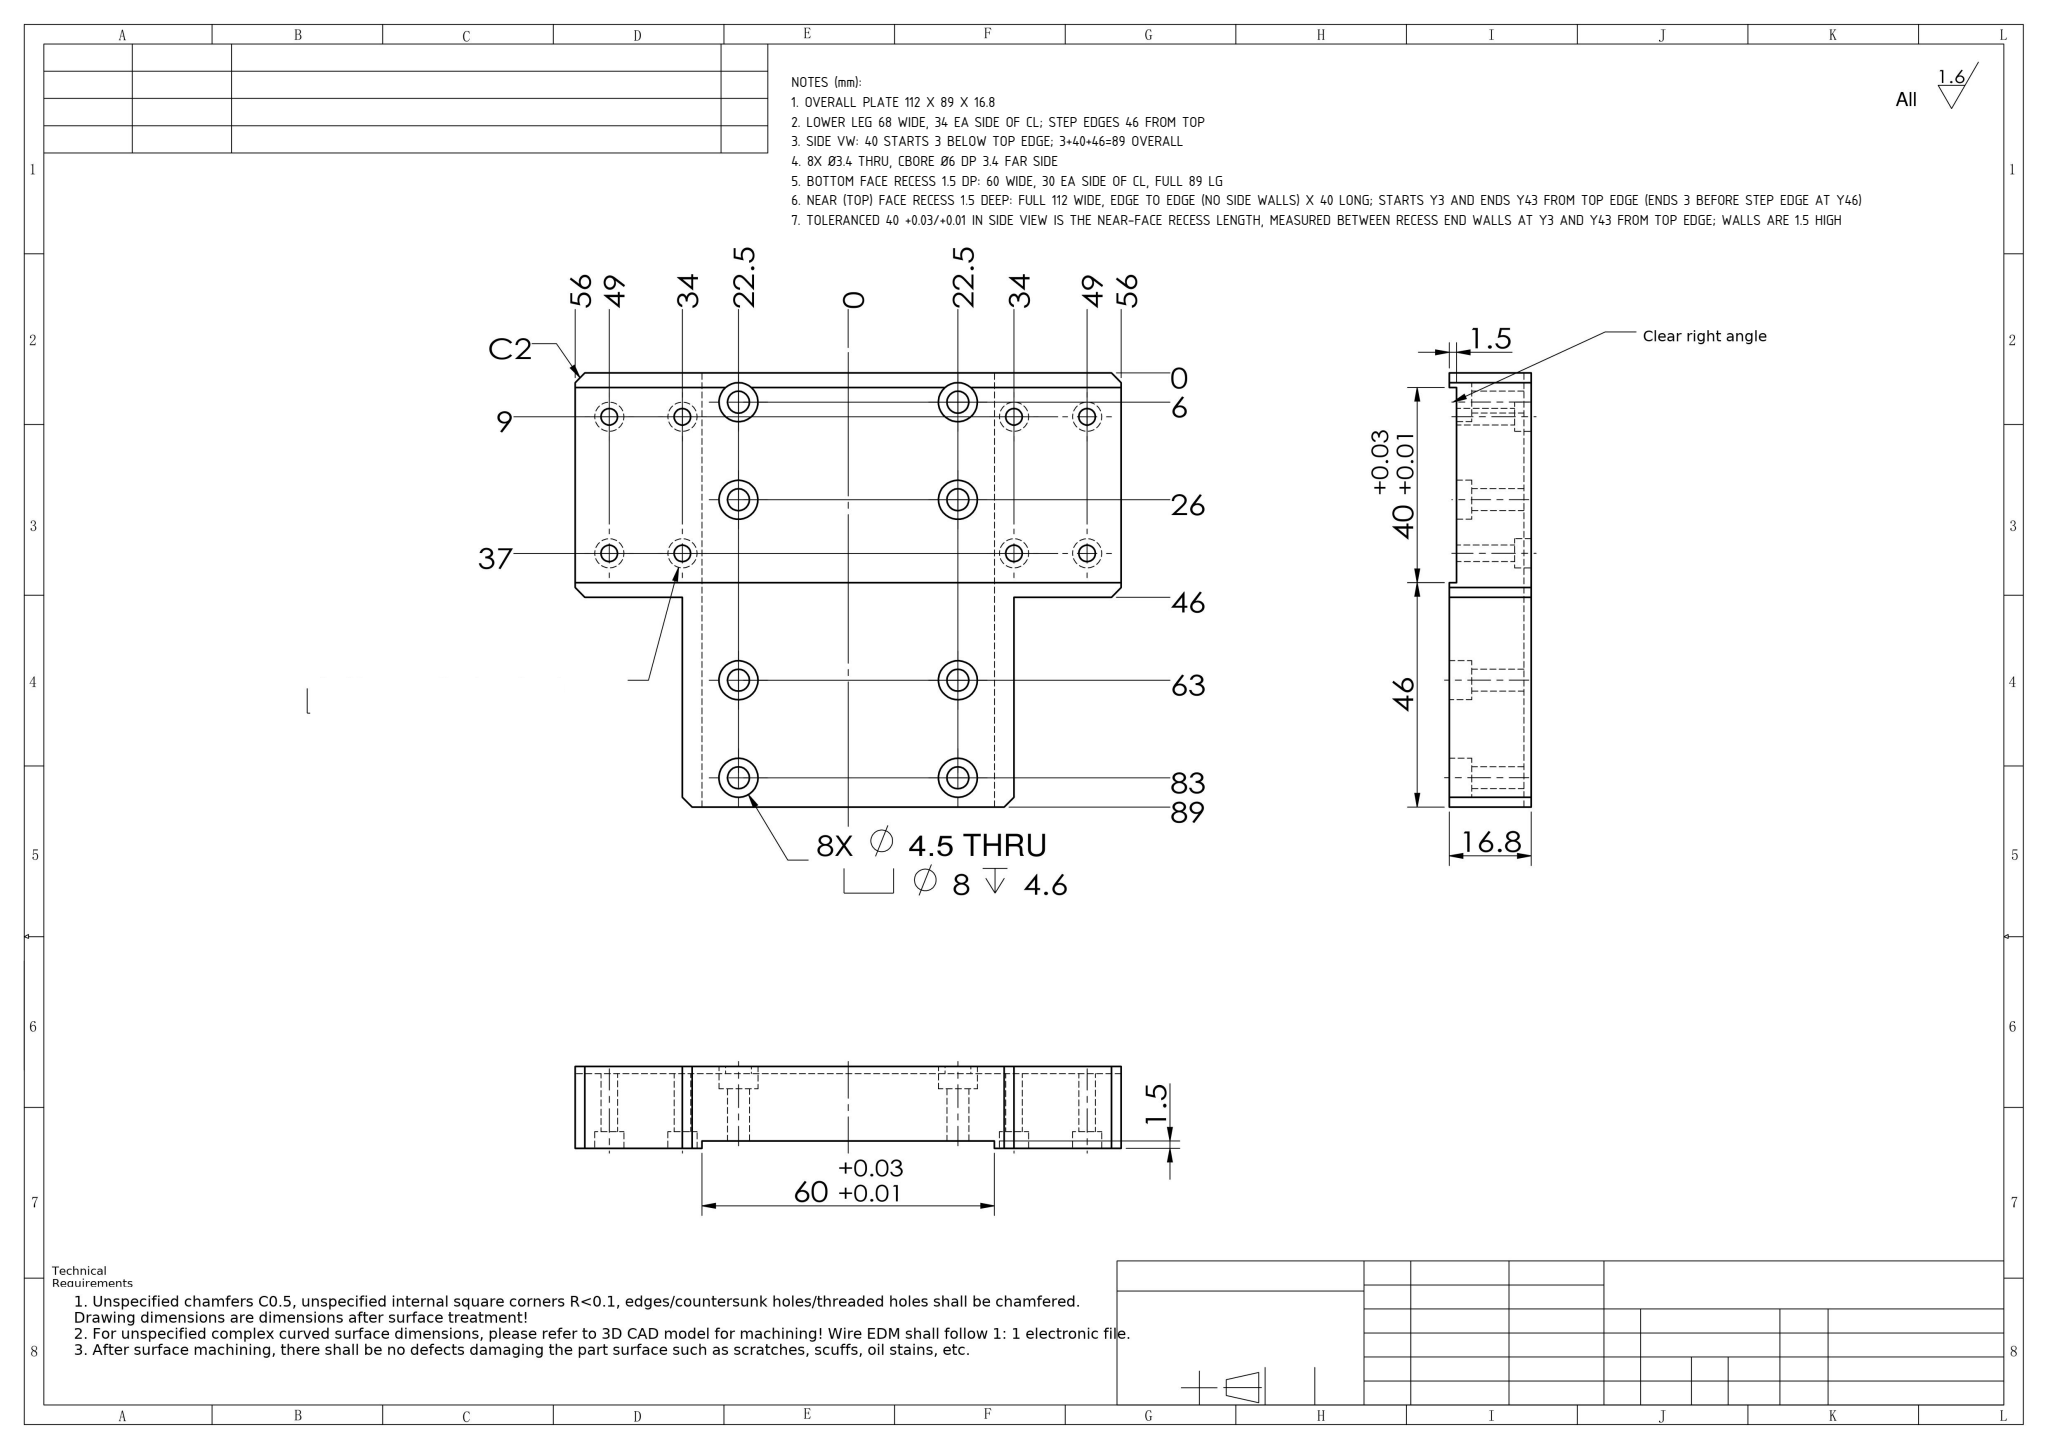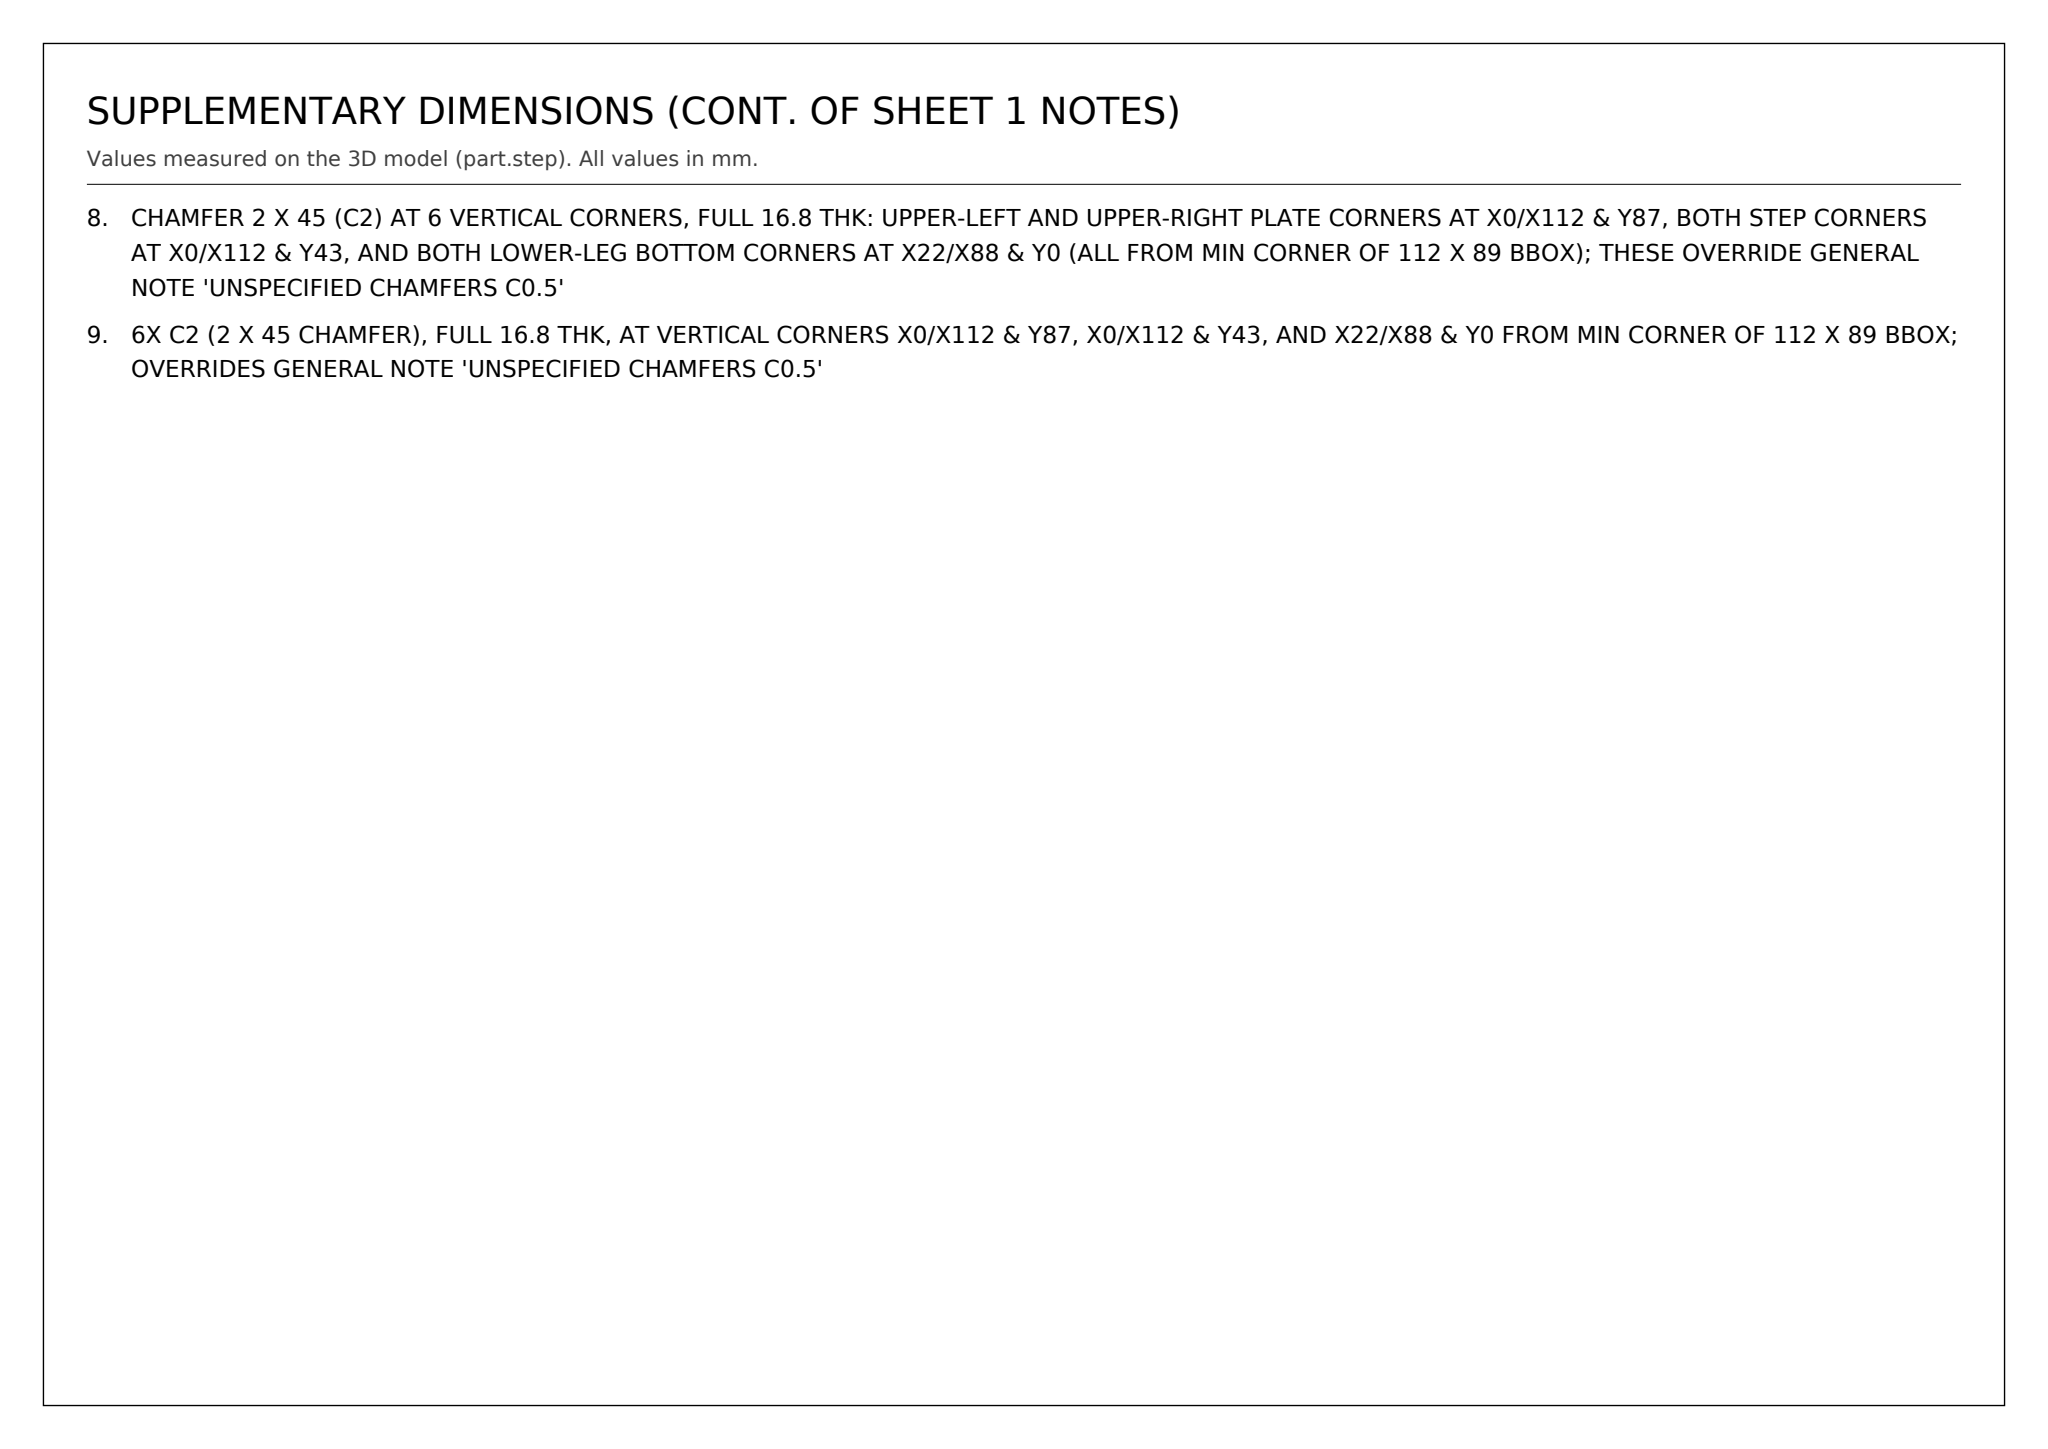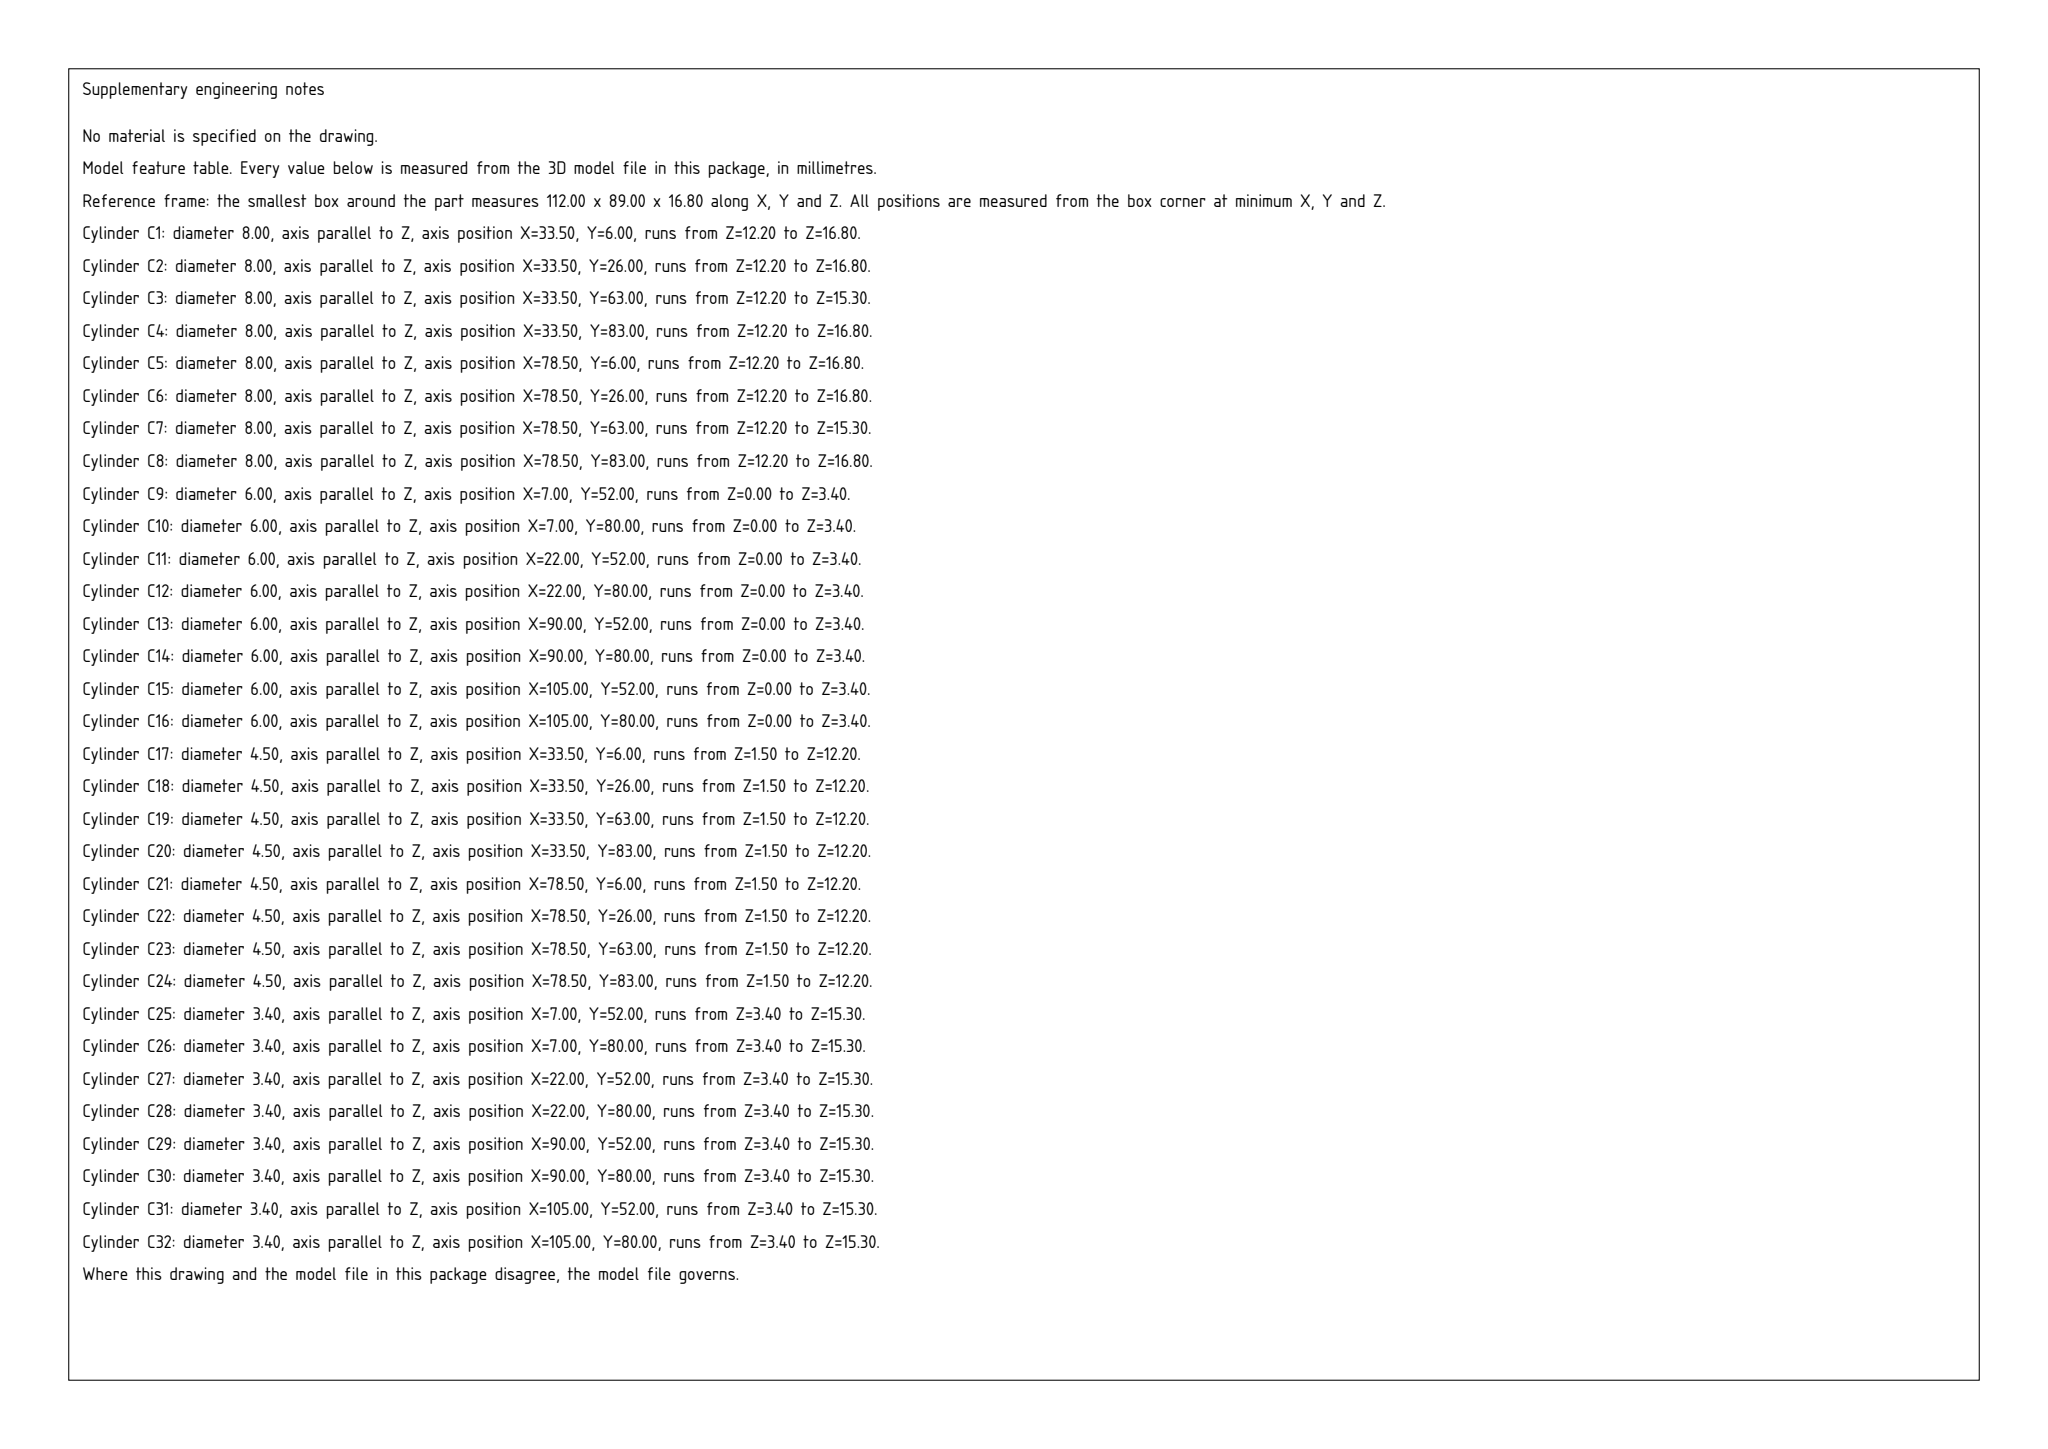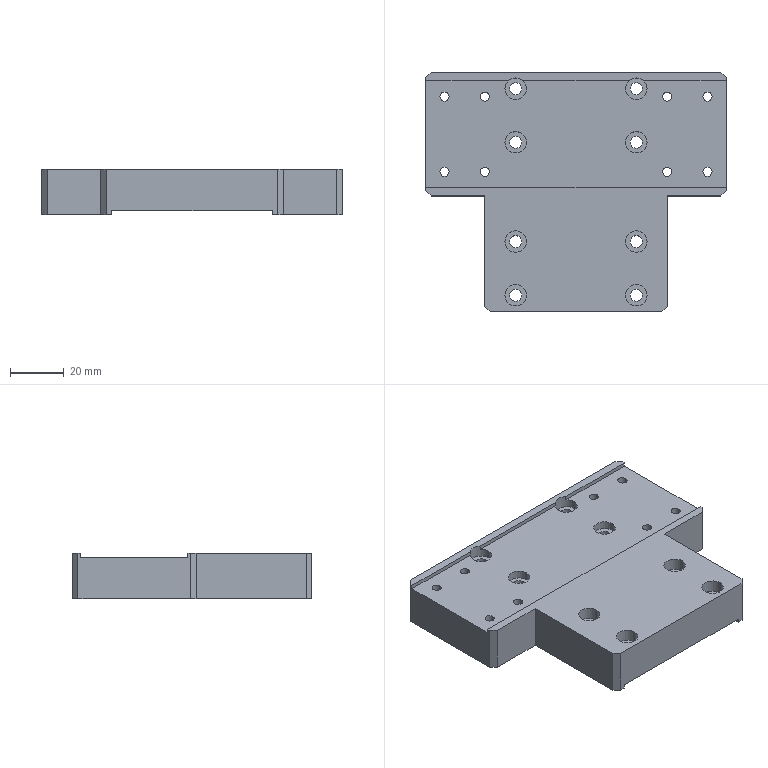Part | SolidWorks | mm | 1 solid | 106 faces | box 112 x 89 x 16.8 mm | volume 116191 mm3 | cylinder 64 | plane 42 | commonest cylinder face diameters 6 x16 3.4 x16 8 x16 4.5 x16
Drawing notes:
OVERALL PLATE 112 X 89 X 16.8 | from the solid: bbox_xyz [112.0, 89.0, 16.8]
LOWER LEG 68 WIDE, 34 EA SIDE OF CL; STEP EDGES 46 FROM TOP | from the solid: Leg side faces are planes x=22.0 and x=90.0, each spanning y[2,43] over full z[0,16.8] -> leg width 90-22 = 68, symmetric about CL at x=56 (34 each side). Step walls are planes y=43 at x[2,22] and x[90,110], i.e. 89-43 = 46 from the top edge.
SIDE VW: 40 STARTS 3 BELOW TOP EDGE; 3+40+46=89 OVERALL | from the solid: y-planes 89, 86, 46, 0: 89-86=3, 86-46=40, 46-0=46
8X Ø3.4 THRU, CBORE Ø6 DP 3.4 FAR SIDE | from the solid: Ø3.4 z-axis L=11.9 at (7/22/90/105 x 52/80); coaxial Ø6 L=3.4 from z=0 face
BOTTOM FACE RECESS 1.5 DP: 60 WIDE, 30 EA SIDE OF CL, FULL 89 LG | from the solid: z=0 face split in 2 lands by floor plane z=1.5 (1.5 deep); recess bounded by x=26 and x=86 planes (60 wide) on 112 bbox (CL at 56), running full 89 in Y
NEAR (TOP) FACE RECESS 1.5 DEEP: FULL 112 WIDE, EDGE TO EDGE (NO SIDE WALLS) X 40 LONG; STARTS Y3 AND ENDS Y43 FROM TOP EDGE (ENDS 3 BEFORE STEP EDGE AT Y46) | from the solid: z=15.3 plane extent x[0,112], y[46,86] between z=16.8 planes y[0,46] and y[86,89] (bbox z 16.8; 16.8-15.3=1.5)
TOLERANCED 40 +0.03/+0.01 IN SIDE VIEW IS THE NEAR-FACE RECESS LENGTH, MEASURED BETWEEN RECESS END WALLS AT Y3 AND Y43 FROM TOP EDGE; WALLS ARE 1.5 HIGH | from the solid: plane y=86 (z 15.3-16.8) and plane y=46 (x 0-112, z 15.3-16.8) are 40 apart; 89-86=3, 89-46=43
CHAMFER 2 X 45 (C2) AT 6 VERTICAL CORNERS, FULL 16.8 THK: UPPER-LEFT AND UPPER-RIGHT PLATE CORNERS AT X0/X112 & Y87, BOTH STEP CORNERS AT X0/X112 & Y43, AND BOTH LOWER-LEG BOTTOM CORNERS AT X22/X88 & Y0 (ALL FROM MIN CORNER OF 112 X 89 BBOX); THESE OVERRIDE GENERAL NOTE 'UNSPECIFIED CHAMFERS C0.5' | from the solid: inclined_planes: six 45/45/90 faces, size [2.0,2.0,16.8], bbox_from [0,43,0], [0,87,0], [110,43,0], [110,87,0], [22,0,0], [88,0,0]
6X C2 (2 X 45 CHAMFER), FULL 16.8 THK, AT VERTICAL CORNERS X0/X112 & Y87, X0/X112 & Y43, AND X22/X88 & Y0 FROM MIN CORNER OF 112 X 89 BBOX; OVERRIDES GENERAL NOTE 'UNSPECIFIED CHAMFERS C0.5' | from the solid: inclined_planes: six 45/45/90 faces, size 2.0 x 2.0 x 16.8, bbox_from [0,43,0], [0,87,0], [110,43,0], [110,87,0], [22,0,0], [88,0,0]
build123d program:
from build123d import *

# Parameters (mm, degrees)
BOSS_EXTRUDE1_DEPTH                               = 16.8
SKETCH2_W                                         = 60
SKETCH2_H                                         = 1.5
CUT_EXTRUDE1_DEPTH                                = 107.486
SKETCH3_W                                         = 1.5
SKETCH3_H                                         = 40
CUT_EXTRUDE2_DEPTH                                = 122.682
HOLE_SIZE_ACCORDING_TO_TYPE_1_HEXAGON_D           = 4.5
HOLE_SIZE_ACCORDING_TO_TYPE_1_HEXAGON_CBORE_D     = 8
HOLE_SIZE_ACCORDING_TO_TYPE_1_HEXAGON_CBORE_DEPTH = 4.6
HOLE_SIZE_ACCORDING_TO_TYPE_0_HEXAGON_D           = 3.4
HOLE_SIZE_ACCORDING_TO_TYPE_0_HEXAGON_CBORE_D     = 6
HOLE_SIZE_ACCORDING_TO_TYPE_0_HEXAGON_CBORE_DEPTH = 3.4
CHAMFER1_SIZE                                     = 2


with BuildPart() as part:
    # Sketch1 → Boss-Extrude1 (new body)
    with BuildSketch(Plane.XY):
        Polygon((-56, -1.5), (-34, -1.5), (-34, -44.5), (34, -44.5), (34, -1.5), (56, -1.5), (56, 44.5), (-56, 44.5), align=None)
    extrude(amount=BOSS_EXTRUDE1_DEPTH)

    # Sketch2 → Cut-Extrude1 (cut, through all)
    with BuildSketch(Plane(origin=(0, 44.5, 0), x_dir=(1, 0, 0), z_dir=(0, 1, 0))):
        with Locations((0, -0.75)):
            Rectangle(SKETCH2_W, SKETCH2_H)
    extrude(amount=-CUT_EXTRUDE1_DEPTH, mode=Mode.SUBTRACT)

    # Sketch3 → Cut-Extrude2 (cut, through all)
    with BuildSketch(Plane.ZY.offset(56)):
        with Locations((16.05, 21.5)):
            Rectangle(SKETCH3_W, SKETCH3_H)
    extrude(amount=-CUT_EXTRUDE2_DEPTH, mode=Mode.SUBTRACT)

    # Hole Size _ according to_ Type 1 Hexagon (through all)
    with Locations(Plane.XY.offset(16.8)):
        with Locations((22.5, 38.5), (-22.5, 38.5), (-22.5, 18.5), (22.5, 18.5), (22.5, -18.5), (22.5, -38.5), (-22.5, -38.5), (-22.5, -18.5)):
            CounterBoreHole(HOLE_SIZE_ACCORDING_TO_TYPE_1_HEXAGON_D / 2, HOLE_SIZE_ACCORDING_TO_TYPE_1_HEXAGON_CBORE_D / 2, HOLE_SIZE_ACCORDING_TO_TYPE_1_HEXAGON_CBORE_DEPTH)

    # Hole Size _ according to_ Type 0 Hexagon (through all)
    with Locations(Plane(origin=(0, 0, 0), x_dir=(-1, 0, 0), z_dir=(0, 0, -1))):
        with Locations((49, 35.5), (34, 35.5), (34, 7.5), (49, 7.5), (-49, 7.5), (-34, 7.5), (-34, 35.5), (-49, 35.5)):
            CounterBoreHole(HOLE_SIZE_ACCORDING_TO_TYPE_0_HEXAGON_D / 2, HOLE_SIZE_ACCORDING_TO_TYPE_0_HEXAGON_CBORE_D / 2, HOLE_SIZE_ACCORDING_TO_TYPE_0_HEXAGON_CBORE_DEPTH)

    # Chamfer1
    chamfer1_edges = [part.edges().sort_by_distance(p)[0] for p in [
        (-56, 44.5, 8.4),
        (56, 44.5, 8.4),
        (56, -1.5, 8.4),
        (34, -44.5, 8.4),
        (-34, -44.5, 8.4),
        (-56, -1.5, 8.4),
    ]]
    chamfer(chamfer1_edges, length=CHAMFER1_SIZE)


solid = part.part